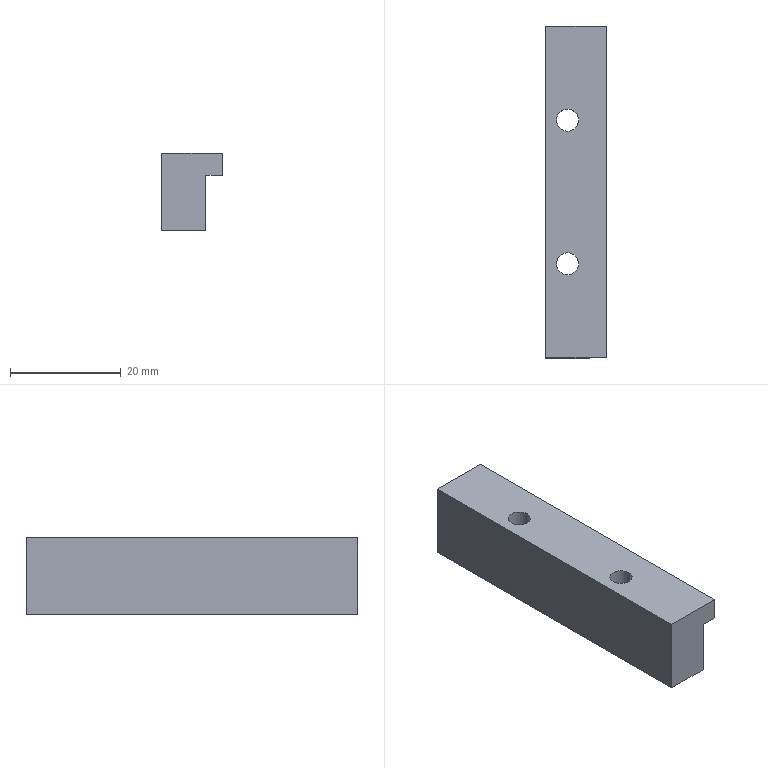Component | NX | 3_RECTANGULAR_GUIDE | 1 solid | 14 faces | box 11 x 60 x 14 mm | volume 6744 mm3 | plane 8 | cylinder 4 | cone 2 | commonest cylinder face diameters 4.2 x2 4 x2
STEP:
#1=CARTESIAN_POINT('',(0.,0.,0.));
#2=DIRECTION('',(0.,0.,1.));
#3=DIRECTION('',(1.,0.,0.));
#4=AXIS2_PLACEMENT_3D('',#1,#2,#3);
#5=CARTESIAN_POINT('',(20.,13.,28.));
#6=VERTEX_POINT('',#5);
#7=CARTESIAN_POINT('',(16.,13.,28.));
#8=VERTEX_POINT('',#7);
#9=CARTESIAN_POINT('',(18.,13.,28.));
#10=DIRECTION('',(0.,0.,-1.));
#11=DIRECTION('',(1.,0.,0.));
#12=AXIS2_PLACEMENT_3D('',#9,#10,#11);
#13=CIRCLE('',#12,2.);
#14=CARTESIAN_POINT('',(25.,-30.,28.));
#15=DIRECTION('',(0.,0.,-1.));
#16=DIRECTION('',(1.,0.,0.));
#17=AXIS2_PLACEMENT_3D('',#14,#15,#16);
#18=PLANE('',#17);
#19=CARTESIAN_POINT('',(-7.,-43.));
#20=DIRECTION('',(1.,0.));
#21=AXIS2_PLACEMENT_2D('',#19,#20);
#22=CIRCLE('',#21,2.);
#23=(GEOMETRIC_REPRESENTATION_CONTEXT(2)PARAMETRIC_REPRESENTATION_CONTEXT()REPRESENTATION_CONTEXT('',''));
#24=DEFINITIONAL_REPRESENTATION('',(#22),#23);
#25=PCURVE('',#18,#24);
#26=CARTESIAN_POINT('',(18.,13.,14.));
#27=DIRECTION('',(-0.,0.,1.));
#28=DIRECTION('',(-1.,0.,-0.));
#29=AXIS2_PLACEMENT_3D('',#26,#27,#28);
#30=CYLINDRICAL_SURFACE('',#29,2.);
#31=CARTESIAN_POINT('',(3.142,14.));
#32=DIRECTION('',(-1.,0.));
#33=VECTOR('',#32,1.);
#34=LINE('',#31,#33);
#35=(GEOMETRIC_REPRESENTATION_CONTEXT(2)PARAMETRIC_REPRESENTATION_CONTEXT()REPRESENTATION_CONTEXT('',''));
#36=DEFINITIONAL_REPRESENTATION('',(#34),#35);
#37=PCURVE('',#30,#36);
#38=SURFACE_CURVE('',#13,(#25,#37),.PCURVE_S1.);
#39=EDGE_CURVE('',#6,#8,#38,.T.);
#40=ORIENTED_EDGE('',*,*,#39,.T.);
#41=CARTESIAN_POINT('',(18.,13.,28.));
#42=DIRECTION('',(0.,0.,-1.));
#43=DIRECTION('',(1.,0.,0.));
#44=AXIS2_PLACEMENT_3D('',#41,#42,#43);
#45=CIRCLE('',#44,2.);
#46=CARTESIAN_POINT('',(-7.,-43.));
#47=DIRECTION('',(1.,0.));
#48=AXIS2_PLACEMENT_2D('',#46,#47);
#49=CIRCLE('',#48,2.);
#50=(GEOMETRIC_REPRESENTATION_CONTEXT(2)PARAMETRIC_REPRESENTATION_CONTEXT()REPRESENTATION_CONTEXT('',''));
#51=DEFINITIONAL_REPRESENTATION('',(#49),#50);
#52=PCURVE('',#18,#51);
#53=CARTESIAN_POINT('',(9.425,14.));
#54=DIRECTION('',(-1.,0.));
#55=VECTOR('',#54,1.);
#56=LINE('',#53,#55);
#57=(GEOMETRIC_REPRESENTATION_CONTEXT(2)PARAMETRIC_REPRESENTATION_CONTEXT()REPRESENTATION_CONTEXT('',''));
#58=DEFINITIONAL_REPRESENTATION('',(#56),#57);
#59=PCURVE('',#30,#58);
#60=SURFACE_CURVE('',#45,(#52,#59),.PCURVE_S1.);
#61=EDGE_CURVE('',#8,#6,#60,.T.);
#62=ORIENTED_EDGE('',*,*,#61,.T.);
#63=EDGE_LOOP('',(#40,#62));
#64=FACE_BOUND('',#63,.T.);
#65=CARTESIAN_POINT('',(20.,-13.,28.));
#66=VERTEX_POINT('',#65);
#67=CARTESIAN_POINT('',(16.,-13.,28.));
#68=VERTEX_POINT('',#67);
#69=CARTESIAN_POINT('',(18.,-13.,28.));
#70=DIRECTION('',(0.,0.,-1.));
#71=DIRECTION('',(1.,0.,0.));
#72=AXIS2_PLACEMENT_3D('',#69,#70,#71);
#73=CIRCLE('',#72,2.);
#74=CARTESIAN_POINT('',(-7.,-17.));
#75=DIRECTION('',(1.,0.));
#76=AXIS2_PLACEMENT_2D('',#74,#75);
#77=CIRCLE('',#76,2.);
#78=(GEOMETRIC_REPRESENTATION_CONTEXT(2)PARAMETRIC_REPRESENTATION_CONTEXT()REPRESENTATION_CONTEXT('',''));
#79=DEFINITIONAL_REPRESENTATION('',(#77),#78);
#80=PCURVE('',#18,#79);
#81=CARTESIAN_POINT('',(18.,-13.,14.));
#82=DIRECTION('',(-0.,0.,1.));
#83=DIRECTION('',(-1.,0.,-0.));
#84=AXIS2_PLACEMENT_3D('',#81,#82,#83);
#85=CYLINDRICAL_SURFACE('',#84,2.);
#86=CARTESIAN_POINT('',(3.142,14.));
#87=DIRECTION('',(-1.,0.));
#88=VECTOR('',#87,1.);
#89=LINE('',#86,#88);
#90=(GEOMETRIC_REPRESENTATION_CONTEXT(2)PARAMETRIC_REPRESENTATION_CONTEXT()REPRESENTATION_CONTEXT('',''));
#91=DEFINITIONAL_REPRESENTATION('',(#89),#90);
#92=PCURVE('',#85,#91);
#93=SURFACE_CURVE('',#73,(#80,#92),.PCURVE_S1.);
#94=EDGE_CURVE('',#66,#68,#93,.T.);
#95=ORIENTED_EDGE('',*,*,#94,.T.);
#96=CARTESIAN_POINT('',(18.,-13.,28.));
#97=DIRECTION('',(0.,0.,-1.));
#98=DIRECTION('',(1.,0.,0.));
#99=AXIS2_PLACEMENT_3D('',#96,#97,#98);
#100=CIRCLE('',#99,2.);
#101=CARTESIAN_POINT('',(-7.,-17.));
#102=DIRECTION('',(1.,0.));
#103=AXIS2_PLACEMENT_2D('',#101,#102);
#104=CIRCLE('',#103,2.);
#105=(GEOMETRIC_REPRESENTATION_CONTEXT(2)PARAMETRIC_REPRESENTATION_CONTEXT()REPRESENTATION_CONTEXT('',''));
#106=DEFINITIONAL_REPRESENTATION('',(#104),#105);
#107=PCURVE('',#18,#106);
#108=CARTESIAN_POINT('',(9.425,14.));
#109=DIRECTION('',(-1.,0.));
#110=VECTOR('',#109,1.);
#111=LINE('',#108,#110);
#112=(GEOMETRIC_REPRESENTATION_CONTEXT(2)PARAMETRIC_REPRESENTATION_CONTEXT()REPRESENTATION_CONTEXT('',''));
#113=DEFINITIONAL_REPRESENTATION('',(#111),#112);
#114=PCURVE('',#85,#113);
#115=SURFACE_CURVE('',#100,(#107,#114),.PCURVE_S1.);
#116=EDGE_CURVE('',#68,#66,#115,.T.);
#117=ORIENTED_EDGE('',*,*,#116,.T.);
#118=EDGE_LOOP('',(#95,#117));
#119=FACE_BOUND('',#118,.T.);
#120=CARTESIAN_POINT('',(25.,30.,28.));
#121=VERTEX_POINT('',#120);
#122=CARTESIAN_POINT('',(14.,30.,28.));
#123=VERTEX_POINT('',#122);
#124=CARTESIAN_POINT('',(25.,30.,28.));
#125=DIRECTION('',(-1.,0.,0.));
#126=VECTOR('',#125,1.);
#127=LINE('',#124,#126);
#128=CARTESIAN_POINT('',(0.,-60.));
#129=DIRECTION('',(-1.,0.));
#130=VECTOR('',#129,1.);
#131=LINE('',#128,#130);
#132=(GEOMETRIC_REPRESENTATION_CONTEXT(2)PARAMETRIC_REPRESENTATION_CONTEXT()REPRESENTATION_CONTEXT('',''));
#133=DEFINITIONAL_REPRESENTATION('',(#131),#132);
#134=PCURVE('',#18,#133);
#135=CARTESIAN_POINT('',(14.,30.,28.));
#136=DIRECTION('',(0.,-1.,0.));
#137=DIRECTION('',(-1.,0.,0.));
#138=AXIS2_PLACEMENT_3D('',#135,#136,#137);
#139=PLANE('',#138);
#140=CARTESIAN_POINT('',(-11.,0.));
#141=DIRECTION('',(1.,0.));
#142=VECTOR('',#141,1.);
#143=LINE('',#140,#142);
#144=(GEOMETRIC_REPRESENTATION_CONTEXT(2)PARAMETRIC_REPRESENTATION_CONTEXT()REPRESENTATION_CONTEXT('',''));
#145=DEFINITIONAL_REPRESENTATION('',(#143),#144);
#146=PCURVE('',#139,#145);
#147=SURFACE_CURVE('',#127,(#134,#146),.PCURVE_S1.);
#148=EDGE_CURVE('',#121,#123,#147,.T.);
#149=ORIENTED_EDGE('',*,*,#148,.T.);
#150=CARTESIAN_POINT('',(14.,-30.,28.));
#151=VERTEX_POINT('',#150);
#152=CARTESIAN_POINT('',(14.,-30.,28.));
#153=DIRECTION('',(0.,1.,0.));
#154=VECTOR('',#153,1.);
#155=LINE('',#152,#154);
#156=CARTESIAN_POINT('',(-11.,0.));
#157=DIRECTION('',(0.,-1.));
#158=VECTOR('',#157,1.);
#159=LINE('',#156,#158);
#160=(GEOMETRIC_REPRESENTATION_CONTEXT(2)PARAMETRIC_REPRESENTATION_CONTEXT()REPRESENTATION_CONTEXT('',''));
#161=DEFINITIONAL_REPRESENTATION('',(#159),#160);
#162=PCURVE('',#18,#161);
#163=CARTESIAN_POINT('',(14.,-30.,24.));
#164=DIRECTION('',(1.,0.,0.));
#165=DIRECTION('',(0.,-1.,0.));
#166=AXIS2_PLACEMENT_3D('',#163,#164,#165);
#167=PLANE('',#166);
#168=CARTESIAN_POINT('',(0.,-4.));
#169=DIRECTION('',(-1.,0.));
#170=VECTOR('',#169,1.);
#171=LINE('',#168,#170);
#172=(GEOMETRIC_REPRESENTATION_CONTEXT(2)PARAMETRIC_REPRESENTATION_CONTEXT()REPRESENTATION_CONTEXT('',''));
#173=DEFINITIONAL_REPRESENTATION('',(#171),#172);
#174=PCURVE('',#167,#173);
#175=SURFACE_CURVE('',#155,(#162,#174),.PCURVE_S1.);
#176=EDGE_CURVE('',#151,#123,#175,.T.);
#177=ORIENTED_EDGE('',*,*,#176,.F.);
#178=CARTESIAN_POINT('',(25.,-30.,28.));
#179=VERTEX_POINT('',#178);
#180=CARTESIAN_POINT('',(25.,-30.,28.));
#181=DIRECTION('',(-1.,0.,0.));
#182=VECTOR('',#181,1.);
#183=LINE('',#180,#182);
#184=CARTESIAN_POINT('',(0.,0.));
#185=DIRECTION('',(-1.,0.));
#186=VECTOR('',#185,1.);
#187=LINE('',#184,#186);
#188=(GEOMETRIC_REPRESENTATION_CONTEXT(2)PARAMETRIC_REPRESENTATION_CONTEXT()REPRESENTATION_CONTEXT('',''));
#189=DEFINITIONAL_REPRESENTATION('',(#187),#188);
#190=PCURVE('',#18,#189);
#191=CARTESIAN_POINT('',(14.,-30.,28.));
#192=DIRECTION('',(0.,-1.,0.));
#193=DIRECTION('',(-1.,0.,0.));
#194=AXIS2_PLACEMENT_3D('',#191,#192,#193);
#195=PLANE('',#194);
#196=CARTESIAN_POINT('',(-11.,0.));
#197=DIRECTION('',(1.,0.));
#198=VECTOR('',#197,1.);
#199=LINE('',#196,#198);
#200=(GEOMETRIC_REPRESENTATION_CONTEXT(2)PARAMETRIC_REPRESENTATION_CONTEXT()REPRESENTATION_CONTEXT('',''));
#201=DEFINITIONAL_REPRESENTATION('',(#199),#200);
#202=PCURVE('',#195,#201);
#203=SURFACE_CURVE('',#183,(#190,#202),.PCURVE_S1.);
#204=EDGE_CURVE('',#179,#151,#203,.T.);
#205=ORIENTED_EDGE('',*,*,#204,.F.);
#206=CARTESIAN_POINT('',(25.,-30.,28.));
#207=DIRECTION('',(0.,1.,0.));
#208=VECTOR('',#207,1.);
#209=LINE('',#206,#208);
#210=CARTESIAN_POINT('',(0.,0.));
#211=DIRECTION('',(0.,-1.));
#212=VECTOR('',#211,1.);
#213=LINE('',#210,#212);
#214=(GEOMETRIC_REPRESENTATION_CONTEXT(2)PARAMETRIC_REPRESENTATION_CONTEXT()REPRESENTATION_CONTEXT('',''));
#215=DEFINITIONAL_REPRESENTATION('',(#213),#214);
#216=PCURVE('',#18,#215);
#217=CARTESIAN_POINT('',(25.,-30.,24.));
#218=DIRECTION('',(-1.,0.,0.));
#219=DIRECTION('',(0.,1.,0.));
#220=AXIS2_PLACEMENT_3D('',#217,#218,#219);
#221=PLANE('',#220);
#222=CARTESIAN_POINT('',(0.,-4.));
#223=DIRECTION('',(1.,0.));
#224=VECTOR('',#223,1.);
#225=LINE('',#222,#224);
#226=(GEOMETRIC_REPRESENTATION_CONTEXT(2)PARAMETRIC_REPRESENTATION_CONTEXT()REPRESENTATION_CONTEXT('',''));
#227=DEFINITIONAL_REPRESENTATION('',(#225),#226);
#228=PCURVE('',#221,#227);
#229=SURFACE_CURVE('',#209,(#216,#228),.PCURVE_S1.);
#230=EDGE_CURVE('',#179,#121,#229,.T.);
#231=ORIENTED_EDGE('',*,*,#230,.T.);
#232=EDGE_LOOP('',(#149,#177,#205,#231));
#233=FACE_BOUND('',#232,.T.);
#234=ADVANCED_FACE('',(#64,#119,#233),#18,.F.);
#235=CARTESIAN_POINT('',(14.,30.,14.));
#236=VERTEX_POINT('',#235);
#237=CARTESIAN_POINT('',(14.,30.,24.));
#238=DIRECTION('',(0.,0.,-1.));
#239=VECTOR('',#238,1.);
#240=LINE('',#237,#239);
#241=CARTESIAN_POINT('',(-60.,0.));
#242=DIRECTION('',(0.,1.));
#243=VECTOR('',#242,1.);
#244=LINE('',#241,#243);
#245=(GEOMETRIC_REPRESENTATION_CONTEXT(2)PARAMETRIC_REPRESENTATION_CONTEXT()REPRESENTATION_CONTEXT('',''));
#246=DEFINITIONAL_REPRESENTATION('',(#244),#245);
#247=PCURVE('',#167,#246);
#248=CARTESIAN_POINT('',(0.,4.));
#249=DIRECTION('',(0.,1.));
#250=VECTOR('',#249,1.);
#251=LINE('',#248,#250);
#252=(GEOMETRIC_REPRESENTATION_CONTEXT(2)PARAMETRIC_REPRESENTATION_CONTEXT()REPRESENTATION_CONTEXT('',''));
#253=DEFINITIONAL_REPRESENTATION('',(#251),#252);
#254=PCURVE('',#139,#253);
#255=SURFACE_CURVE('',#240,(#247,#254),.PCURVE_S1.);
#256=EDGE_CURVE('',#123,#236,#255,.T.);
#257=ORIENTED_EDGE('',*,*,#256,.T.);
#258=CARTESIAN_POINT('',(14.,-30.,14.));
#259=VERTEX_POINT('',#258);
#260=CARTESIAN_POINT('',(14.,-30.,14.));
#261=DIRECTION('',(0.,1.,0.));
#262=VECTOR('',#261,1.);
#263=LINE('',#260,#262);
#264=CARTESIAN_POINT('',(0.,10.));
#265=DIRECTION('',(-1.,0.));
#266=VECTOR('',#265,1.);
#267=LINE('',#264,#266);
#268=(GEOMETRIC_REPRESENTATION_CONTEXT(2)PARAMETRIC_REPRESENTATION_CONTEXT()REPRESENTATION_CONTEXT('',''));
#269=DEFINITIONAL_REPRESENTATION('',(#267),#268);
#270=PCURVE('',#167,#269);
#271=CARTESIAN_POINT('',(14.,-30.,14.));
#272=DIRECTION('',(-0.,0.,1.));
#273=DIRECTION('',(-1.,0.,-0.));
#274=AXIS2_PLACEMENT_3D('',#271,#272,#273);
#275=PLANE('',#274);
#276=CARTESIAN_POINT('',(0.,0.));
#277=DIRECTION('',(0.,-1.));
#278=VECTOR('',#277,1.);
#279=LINE('',#276,#278);
#280=(GEOMETRIC_REPRESENTATION_CONTEXT(2)PARAMETRIC_REPRESENTATION_CONTEXT()REPRESENTATION_CONTEXT('',''));
#281=DEFINITIONAL_REPRESENTATION('',(#279),#280);
#282=PCURVE('',#275,#281);
#283=SURFACE_CURVE('',#263,(#270,#282),.PCURVE_S1.);
#284=EDGE_CURVE('',#259,#236,#283,.T.);
#285=ORIENTED_EDGE('',*,*,#284,.F.);
#286=CARTESIAN_POINT('',(14.,-30.,28.));
#287=DIRECTION('',(0.,0.,-1.));
#288=VECTOR('',#287,1.);
#289=LINE('',#286,#288);
#290=CARTESIAN_POINT('',(0.,-4.));
#291=DIRECTION('',(0.,1.));
#292=VECTOR('',#291,1.);
#293=LINE('',#290,#292);
#294=(GEOMETRIC_REPRESENTATION_CONTEXT(2)PARAMETRIC_REPRESENTATION_CONTEXT()REPRESENTATION_CONTEXT('',''));
#295=DEFINITIONAL_REPRESENTATION('',(#293),#294);
#296=PCURVE('',#167,#295);
#297=CARTESIAN_POINT('',(0.,0.));
#298=DIRECTION('',(0.,1.));
#299=VECTOR('',#298,1.);
#300=LINE('',#297,#299);
#301=(GEOMETRIC_REPRESENTATION_CONTEXT(2)PARAMETRIC_REPRESENTATION_CONTEXT()REPRESENTATION_CONTEXT('',''));
#302=DEFINITIONAL_REPRESENTATION('',(#300),#301);
#303=PCURVE('',#195,#302);
#304=SURFACE_CURVE('',#289,(#296,#303),.PCURVE_S1.);
#305=EDGE_CURVE('',#151,#259,#304,.T.);
#306=ORIENTED_EDGE('',*,*,#305,.F.);
#307=ORIENTED_EDGE('',*,*,#176,.T.);
#308=EDGE_LOOP('',(#257,#285,#306,#307));
#309=FACE_BOUND('',#308,.T.);
#310=ADVANCED_FACE('',(#309),#167,.F.);
#311=CARTESIAN_POINT('',(16.,13.,14.));
#312=VERTEX_POINT('',#311);
#313=CARTESIAN_POINT('',(18.,13.,14.));
#314=DIRECTION('',(-0.,0.,1.));
#315=DIRECTION('',(-1.,0.,-0.));
#316=AXIS2_PLACEMENT_3D('',#313,#314,#315);
#317=CIRCLE('',#316,2.);
#318=CARTESIAN_POINT('',(-4.,-43.));
#319=DIRECTION('',(1.,0.));
#320=AXIS2_PLACEMENT_2D('',#318,#319);
#321=CIRCLE('',#320,2.);
#322=(GEOMETRIC_REPRESENTATION_CONTEXT(2)PARAMETRIC_REPRESENTATION_CONTEXT()REPRESENTATION_CONTEXT('',''));
#323=DEFINITIONAL_REPRESENTATION('',(#321),#322);
#324=PCURVE('',#275,#323);
#325=CARTESIAN_POINT('',(0.,0.));
#326=DIRECTION('',(1.,0.));
#327=VECTOR('',#326,1.);
#328=LINE('',#325,#327);
#329=(GEOMETRIC_REPRESENTATION_CONTEXT(2)PARAMETRIC_REPRESENTATION_CONTEXT()REPRESENTATION_CONTEXT('',''));
#330=DEFINITIONAL_REPRESENTATION('',(#328),#329);
#331=PCURVE('',#30,#330);
#332=SURFACE_CURVE('',#317,(#324,#331),.PCURVE_S1.);
#333=EDGE_CURVE('',#312,#312,#332,.T.);
#334=ORIENTED_EDGE('',*,*,#333,.T.);
#335=EDGE_LOOP('',(#334));
#336=FACE_BOUND('',#335,.T.);
#337=CARTESIAN_POINT('',(16.,-13.,14.));
#338=VERTEX_POINT('',#337);
#339=CARTESIAN_POINT('',(18.,-13.,14.));
#340=DIRECTION('',(-0.,0.,1.));
#341=DIRECTION('',(-1.,0.,-0.));
#342=AXIS2_PLACEMENT_3D('',#339,#340,#341);
#343=CIRCLE('',#342,2.);
#344=CARTESIAN_POINT('',(-4.,-17.));
#345=DIRECTION('',(1.,0.));
#346=AXIS2_PLACEMENT_2D('',#344,#345);
#347=CIRCLE('',#346,2.);
#348=(GEOMETRIC_REPRESENTATION_CONTEXT(2)PARAMETRIC_REPRESENTATION_CONTEXT()REPRESENTATION_CONTEXT('',''));
#349=DEFINITIONAL_REPRESENTATION('',(#347),#348);
#350=PCURVE('',#275,#349);
#351=CARTESIAN_POINT('',(0.,0.));
#352=DIRECTION('',(1.,0.));
#353=VECTOR('',#352,1.);
#354=LINE('',#351,#353);
#355=(GEOMETRIC_REPRESENTATION_CONTEXT(2)PARAMETRIC_REPRESENTATION_CONTEXT()REPRESENTATION_CONTEXT('',''));
#356=DEFINITIONAL_REPRESENTATION('',(#354),#355);
#357=PCURVE('',#85,#356);
#358=SURFACE_CURVE('',#343,(#350,#357),.PCURVE_S1.);
#359=EDGE_CURVE('',#338,#338,#358,.T.);
#360=ORIENTED_EDGE('',*,*,#359,.T.);
#361=EDGE_LOOP('',(#360));
#362=FACE_BOUND('',#361,.T.);
#363=CARTESIAN_POINT('',(15.9,22.,14.));
#364=VERTEX_POINT('',#363);
#365=CARTESIAN_POINT('',(18.,22.,14.));
#366=DIRECTION('',(-0.,0.,1.));
#367=DIRECTION('',(-1.,0.,-0.));
#368=AXIS2_PLACEMENT_3D('',#365,#366,#367);
#369=CIRCLE('',#368,2.1);
#370=CARTESIAN_POINT('',(-4.,-52.));
#371=DIRECTION('',(1.,0.));
#372=AXIS2_PLACEMENT_2D('',#370,#371);
#373=CIRCLE('',#372,2.1);
#374=(GEOMETRIC_REPRESENTATION_CONTEXT(2)PARAMETRIC_REPRESENTATION_CONTEXT()REPRESENTATION_CONTEXT('',''));
#375=DEFINITIONAL_REPRESENTATION('',(#373),#374);
#376=PCURVE('',#275,#375);
#377=CARTESIAN_POINT('',(18.,22.,14.));
#378=DIRECTION('',(-0.,0.,1.));
#379=DIRECTION('',(-1.,0.,-0.));
#380=AXIS2_PLACEMENT_3D('',#377,#378,#379);
#381=CYLINDRICAL_SURFACE('',#380,2.1);
#382=CARTESIAN_POINT('',(0.,0.));
#383=DIRECTION('',(1.,0.));
#384=VECTOR('',#383,1.);
#385=LINE('',#382,#384);
#386=(GEOMETRIC_REPRESENTATION_CONTEXT(2)PARAMETRIC_REPRESENTATION_CONTEXT()REPRESENTATION_CONTEXT('',''));
#387=DEFINITIONAL_REPRESENTATION('',(#385),#386);
#388=PCURVE('',#381,#387);
#389=SURFACE_CURVE('',#369,(#376,#388),.PCURVE_S1.);
#390=EDGE_CURVE('',#364,#364,#389,.T.);
#391=ORIENTED_EDGE('',*,*,#390,.T.);
#392=EDGE_LOOP('',(#391));
#393=FACE_BOUND('',#392,.T.);
#394=CARTESIAN_POINT('',(15.9,-22.,14.));
#395=VERTEX_POINT('',#394);
#396=CARTESIAN_POINT('',(18.,-22.,14.));
#397=DIRECTION('',(-0.,0.,1.));
#398=DIRECTION('',(-1.,0.,-0.));
#399=AXIS2_PLACEMENT_3D('',#396,#397,#398);
#400=CIRCLE('',#399,2.1);
#401=CARTESIAN_POINT('',(-4.,-8.));
#402=DIRECTION('',(1.,0.));
#403=AXIS2_PLACEMENT_2D('',#401,#402);
#404=CIRCLE('',#403,2.1);
#405=(GEOMETRIC_REPRESENTATION_CONTEXT(2)PARAMETRIC_REPRESENTATION_CONTEXT()REPRESENTATION_CONTEXT('',''));
#406=DEFINITIONAL_REPRESENTATION('',(#404),#405);
#407=PCURVE('',#275,#406);
#408=CARTESIAN_POINT('',(18.,-22.,14.));
#409=DIRECTION('',(-0.,0.,1.));
#410=DIRECTION('',(-1.,0.,-0.));
#411=AXIS2_PLACEMENT_3D('',#408,#409,#410);
#412=CYLINDRICAL_SURFACE('',#411,2.1);
#413=CARTESIAN_POINT('',(0.,0.));
#414=DIRECTION('',(1.,0.));
#415=VECTOR('',#414,1.);
#416=LINE('',#413,#415);
#417=(GEOMETRIC_REPRESENTATION_CONTEXT(2)PARAMETRIC_REPRESENTATION_CONTEXT()REPRESENTATION_CONTEXT('',''));
#418=DEFINITIONAL_REPRESENTATION('',(#416),#417);
#419=PCURVE('',#412,#418);
#420=SURFACE_CURVE('',#400,(#407,#419),.PCURVE_S1.);
#421=EDGE_CURVE('',#395,#395,#420,.T.);
#422=ORIENTED_EDGE('',*,*,#421,.T.);
#423=EDGE_LOOP('',(#422));
#424=FACE_BOUND('',#423,.T.);
#425=CARTESIAN_POINT('',(22.,30.,14.));
#426=VERTEX_POINT('',#425);
#427=CARTESIAN_POINT('',(14.,30.,14.));
#428=DIRECTION('',(1.,0.,0.));
#429=VECTOR('',#428,1.);
#430=LINE('',#427,#429);
#431=CARTESIAN_POINT('',(0.,-60.));
#432=DIRECTION('',(-1.,0.));
#433=VECTOR('',#432,1.);
#434=LINE('',#431,#433);
#435=(GEOMETRIC_REPRESENTATION_CONTEXT(2)PARAMETRIC_REPRESENTATION_CONTEXT()REPRESENTATION_CONTEXT('',''));
#436=DEFINITIONAL_REPRESENTATION('',(#434),#435);
#437=PCURVE('',#275,#436);
#438=CARTESIAN_POINT('',(0.,14.));
#439=DIRECTION('',(-1.,-0.));
#440=VECTOR('',#439,1.);
#441=LINE('',#438,#440);
#442=(GEOMETRIC_REPRESENTATION_CONTEXT(2)PARAMETRIC_REPRESENTATION_CONTEXT()REPRESENTATION_CONTEXT('',''));
#443=DEFINITIONAL_REPRESENTATION('',(#441),#442);
#444=PCURVE('',#139,#443);
#445=SURFACE_CURVE('',#430,(#437,#444),.PCURVE_S1.);
#446=EDGE_CURVE('',#236,#426,#445,.T.);
#447=ORIENTED_EDGE('',*,*,#446,.T.);
#448=CARTESIAN_POINT('',(22.,-30.,14.));
#449=VERTEX_POINT('',#448);
#450=CARTESIAN_POINT('',(22.,-30.,14.));
#451=DIRECTION('',(0.,1.,0.));
#452=VECTOR('',#451,1.);
#453=LINE('',#450,#452);
#454=CARTESIAN_POINT('',(-8.,0.));
#455=DIRECTION('',(0.,-1.));
#456=VECTOR('',#455,1.);
#457=LINE('',#454,#456);
#458=(GEOMETRIC_REPRESENTATION_CONTEXT(2)PARAMETRIC_REPRESENTATION_CONTEXT()REPRESENTATION_CONTEXT('',''));
#459=DEFINITIONAL_REPRESENTATION('',(#457),#458);
#460=PCURVE('',#275,#459);
#461=CARTESIAN_POINT('',(22.,-30.,14.));
#462=DIRECTION('',(-1.,0.,-0.));
#463=DIRECTION('',(0.,0.,-1.));
#464=AXIS2_PLACEMENT_3D('',#461,#462,#463);
#465=PLANE('',#464);
#466=CARTESIAN_POINT('',(0.,0.));
#467=DIRECTION('',(0.,-1.));
#468=VECTOR('',#467,1.);
#469=LINE('',#466,#468);
#470=(GEOMETRIC_REPRESENTATION_CONTEXT(2)PARAMETRIC_REPRESENTATION_CONTEXT()REPRESENTATION_CONTEXT('',''));
#471=DEFINITIONAL_REPRESENTATION('',(#469),#470);
#472=PCURVE('',#465,#471);
#473=SURFACE_CURVE('',#453,(#460,#472),.PCURVE_S1.);
#474=EDGE_CURVE('',#449,#426,#473,.T.);
#475=ORIENTED_EDGE('',*,*,#474,.F.);
#476=CARTESIAN_POINT('',(14.,-30.,14.));
#477=DIRECTION('',(1.,0.,0.));
#478=VECTOR('',#477,1.);
#479=LINE('',#476,#478);
#480=CARTESIAN_POINT('',(0.,0.));
#481=DIRECTION('',(-1.,0.));
#482=VECTOR('',#481,1.);
#483=LINE('',#480,#482);
#484=(GEOMETRIC_REPRESENTATION_CONTEXT(2)PARAMETRIC_REPRESENTATION_CONTEXT()REPRESENTATION_CONTEXT('',''));
#485=DEFINITIONAL_REPRESENTATION('',(#483),#484);
#486=PCURVE('',#275,#485);
#487=CARTESIAN_POINT('',(0.,14.));
#488=DIRECTION('',(-1.,-0.));
#489=VECTOR('',#488,1.);
#490=LINE('',#487,#489);
#491=(GEOMETRIC_REPRESENTATION_CONTEXT(2)PARAMETRIC_REPRESENTATION_CONTEXT()REPRESENTATION_CONTEXT('',''));
#492=DEFINITIONAL_REPRESENTATION('',(#490),#491);
#493=PCURVE('',#195,#492);
#494=SURFACE_CURVE('',#479,(#486,#493),.PCURVE_S1.);
#495=EDGE_CURVE('',#259,#449,#494,.T.);
#496=ORIENTED_EDGE('',*,*,#495,.F.);
#497=ORIENTED_EDGE('',*,*,#284,.T.);
#498=EDGE_LOOP('',(#447,#475,#496,#497));
#499=FACE_BOUND('',#498,.T.);
#500=ADVANCED_FACE('',(#336,#362,#393,#424,#499),#275,.F.);
#501=CARTESIAN_POINT('',(22.,30.,24.));
#502=VERTEX_POINT('',#501);
#503=CARTESIAN_POINT('',(22.,30.,14.));
#504=DIRECTION('',(-0.,0.,1.));
#505=VECTOR('',#504,1.);
#506=LINE('',#503,#505);
#507=CARTESIAN_POINT('',(0.,-60.));
#508=DIRECTION('',(-1.,0.));
#509=VECTOR('',#508,1.);
#510=LINE('',#507,#509);
#511=(GEOMETRIC_REPRESENTATION_CONTEXT(2)PARAMETRIC_REPRESENTATION_CONTEXT()REPRESENTATION_CONTEXT('',''));
#512=DEFINITIONAL_REPRESENTATION('',(#510),#511);
#513=PCURVE('',#465,#512);
#514=CARTESIAN_POINT('',(-8.,14.));
#515=DIRECTION('',(0.,-1.));
#516=VECTOR('',#515,1.);
#517=LINE('',#514,#516);
#518=(GEOMETRIC_REPRESENTATION_CONTEXT(2)PARAMETRIC_REPRESENTATION_CONTEXT()REPRESENTATION_CONTEXT('',''));
#519=DEFINITIONAL_REPRESENTATION('',(#517),#518);
#520=PCURVE('',#139,#519);
#521=SURFACE_CURVE('',#506,(#513,#520),.PCURVE_S1.);
#522=EDGE_CURVE('',#426,#502,#521,.T.);
#523=ORIENTED_EDGE('',*,*,#522,.T.);
#524=CARTESIAN_POINT('',(22.,-30.,24.));
#525=VERTEX_POINT('',#524);
#526=CARTESIAN_POINT('',(22.,-30.,24.));
#527=DIRECTION('',(0.,1.,0.));
#528=VECTOR('',#527,1.);
#529=LINE('',#526,#528);
#530=CARTESIAN_POINT('',(-10.,0.));
#531=DIRECTION('',(0.,-1.));
#532=VECTOR('',#531,1.);
#533=LINE('',#530,#532);
#534=(GEOMETRIC_REPRESENTATION_CONTEXT(2)PARAMETRIC_REPRESENTATION_CONTEXT()REPRESENTATION_CONTEXT('',''));
#535=DEFINITIONAL_REPRESENTATION('',(#533),#534);
#536=PCURVE('',#465,#535);
#537=CARTESIAN_POINT('',(22.,-30.,24.));
#538=DIRECTION('',(-0.,0.,1.));
#539=DIRECTION('',(-1.,0.,-0.));
#540=AXIS2_PLACEMENT_3D('',#537,#538,#539);
#541=PLANE('',#540);
#542=CARTESIAN_POINT('',(0.,0.));
#543=DIRECTION('',(0.,-1.));
#544=VECTOR('',#543,1.);
#545=LINE('',#542,#544);
#546=(GEOMETRIC_REPRESENTATION_CONTEXT(2)PARAMETRIC_REPRESENTATION_CONTEXT()REPRESENTATION_CONTEXT('',''));
#547=DEFINITIONAL_REPRESENTATION('',(#545),#546);
#548=PCURVE('',#541,#547);
#549=SURFACE_CURVE('',#529,(#536,#548),.PCURVE_S1.);
#550=EDGE_CURVE('',#525,#502,#549,.T.);
#551=ORIENTED_EDGE('',*,*,#550,.F.);
#552=CARTESIAN_POINT('',(22.,-30.,14.));
#553=DIRECTION('',(-0.,0.,1.));
#554=VECTOR('',#553,1.);
#555=LINE('',#552,#554);
#556=CARTESIAN_POINT('',(0.,0.));
#557=DIRECTION('',(-1.,0.));
#558=VECTOR('',#557,1.);
#559=LINE('',#556,#558);
#560=(GEOMETRIC_REPRESENTATION_CONTEXT(2)PARAMETRIC_REPRESENTATION_CONTEXT()REPRESENTATION_CONTEXT('',''));
#561=DEFINITIONAL_REPRESENTATION('',(#559),#560);
#562=PCURVE('',#465,#561);
#563=CARTESIAN_POINT('',(-8.,14.));
#564=DIRECTION('',(0.,-1.));
#565=VECTOR('',#564,1.);
#566=LINE('',#563,#565);
#567=(GEOMETRIC_REPRESENTATION_CONTEXT(2)PARAMETRIC_REPRESENTATION_CONTEXT()REPRESENTATION_CONTEXT('',''));
#568=DEFINITIONAL_REPRESENTATION('',(#566),#567);
#569=PCURVE('',#195,#568);
#570=SURFACE_CURVE('',#555,(#562,#569),.PCURVE_S1.);
#571=EDGE_CURVE('',#449,#525,#570,.T.);
#572=ORIENTED_EDGE('',*,*,#571,.F.);
#573=ORIENTED_EDGE('',*,*,#474,.T.);
#574=EDGE_LOOP('',(#523,#551,#572,#573));
#575=FACE_BOUND('',#574,.T.);
#576=ADVANCED_FACE('',(#575),#465,.F.);
#577=CARTESIAN_POINT('',(25.,30.,24.));
#578=VERTEX_POINT('',#577);
#579=CARTESIAN_POINT('',(22.,30.,24.));
#580=DIRECTION('',(1.,0.,0.));
#581=VECTOR('',#580,1.);
#582=LINE('',#579,#581);
#583=CARTESIAN_POINT('',(0.,-60.));
#584=DIRECTION('',(-1.,0.));
#585=VECTOR('',#584,1.);
#586=LINE('',#583,#585);
#587=(GEOMETRIC_REPRESENTATION_CONTEXT(2)PARAMETRIC_REPRESENTATION_CONTEXT()REPRESENTATION_CONTEXT('',''));
#588=DEFINITIONAL_REPRESENTATION('',(#586),#587);
#589=PCURVE('',#541,#588);
#590=CARTESIAN_POINT('',(-8.,4.));
#591=DIRECTION('',(-1.,-0.));
#592=VECTOR('',#591,1.);
#593=LINE('',#590,#592);
#594=(GEOMETRIC_REPRESENTATION_CONTEXT(2)PARAMETRIC_REPRESENTATION_CONTEXT()REPRESENTATION_CONTEXT('',''));
#595=DEFINITIONAL_REPRESENTATION('',(#593),#594);
#596=PCURVE('',#139,#595);
#597=SURFACE_CURVE('',#582,(#589,#596),.PCURVE_S1.);
#598=EDGE_CURVE('',#502,#578,#597,.T.);
#599=ORIENTED_EDGE('',*,*,#598,.T.);
#600=CARTESIAN_POINT('',(25.,-30.,24.));
#601=VERTEX_POINT('',#600);
#602=CARTESIAN_POINT('',(25.,-30.,24.));
#603=DIRECTION('',(0.,1.,0.));
#604=VECTOR('',#603,1.);
#605=LINE('',#602,#604);
#606=CARTESIAN_POINT('',(-3.,0.));
#607=DIRECTION('',(0.,-1.));
#608=VECTOR('',#607,1.);
#609=LINE('',#606,#608);
#610=(GEOMETRIC_REPRESENTATION_CONTEXT(2)PARAMETRIC_REPRESENTATION_CONTEXT()REPRESENTATION_CONTEXT('',''));
#611=DEFINITIONAL_REPRESENTATION('',(#609),#610);
#612=PCURVE('',#541,#611);
#613=CARTESIAN_POINT('',(0.,0.));
#614=DIRECTION('',(1.,0.));
#615=VECTOR('',#614,1.);
#616=LINE('',#613,#615);
#617=(GEOMETRIC_REPRESENTATION_CONTEXT(2)PARAMETRIC_REPRESENTATION_CONTEXT()REPRESENTATION_CONTEXT('',''));
#618=DEFINITIONAL_REPRESENTATION('',(#616),#617);
#619=PCURVE('',#221,#618);
#620=SURFACE_CURVE('',#605,(#612,#619),.PCURVE_S1.);
#621=EDGE_CURVE('',#601,#578,#620,.T.);
#622=ORIENTED_EDGE('',*,*,#621,.F.);
#623=CARTESIAN_POINT('',(22.,-30.,24.));
#624=DIRECTION('',(1.,0.,0.));
#625=VECTOR('',#624,1.);
#626=LINE('',#623,#625);
#627=CARTESIAN_POINT('',(0.,0.));
#628=DIRECTION('',(-1.,0.));
#629=VECTOR('',#628,1.);
#630=LINE('',#627,#629);
#631=(GEOMETRIC_REPRESENTATION_CONTEXT(2)PARAMETRIC_REPRESENTATION_CONTEXT()REPRESENTATION_CONTEXT('',''));
#632=DEFINITIONAL_REPRESENTATION('',(#630),#631);
#633=PCURVE('',#541,#632);
#634=CARTESIAN_POINT('',(-8.,4.));
#635=DIRECTION('',(-1.,-0.));
#636=VECTOR('',#635,1.);
#637=LINE('',#634,#636);
#638=(GEOMETRIC_REPRESENTATION_CONTEXT(2)PARAMETRIC_REPRESENTATION_CONTEXT()REPRESENTATION_CONTEXT('',''));
#639=DEFINITIONAL_REPRESENTATION('',(#637),#638);
#640=PCURVE('',#195,#639);
#641=SURFACE_CURVE('',#626,(#633,#640),.PCURVE_S1.);
#642=EDGE_CURVE('',#525,#601,#641,.T.);
#643=ORIENTED_EDGE('',*,*,#642,.F.);
#644=ORIENTED_EDGE('',*,*,#550,.T.);
#645=EDGE_LOOP('',(#599,#622,#643,#644));
#646=FACE_BOUND('',#645,.T.);
#647=ADVANCED_FACE('',(#646),#541,.F.);
#648=CARTESIAN_POINT('',(25.,30.,24.));
#649=DIRECTION('',(0.,0.,1.));
#650=VECTOR('',#649,1.);
#651=LINE('',#648,#650);
#652=CARTESIAN_POINT('',(60.,0.));
#653=DIRECTION('',(0.,-1.));
#654=VECTOR('',#653,1.);
#655=LINE('',#652,#654);
#656=(GEOMETRIC_REPRESENTATION_CONTEXT(2)PARAMETRIC_REPRESENTATION_CONTEXT()REPRESENTATION_CONTEXT('',''));
#657=DEFINITIONAL_REPRESENTATION('',(#655),#656);
#658=PCURVE('',#221,#657);
#659=CARTESIAN_POINT('',(-11.,4.));
#660=DIRECTION('',(0.,-1.));
#661=VECTOR('',#660,1.);
#662=LINE('',#659,#661);
#663=(GEOMETRIC_REPRESENTATION_CONTEXT(2)PARAMETRIC_REPRESENTATION_CONTEXT()REPRESENTATION_CONTEXT('',''));
#664=DEFINITIONAL_REPRESENTATION('',(#662),#663);
#665=PCURVE('',#139,#664);
#666=SURFACE_CURVE('',#651,(#658,#665),.PCURVE_S1.);
#667=EDGE_CURVE('',#578,#121,#666,.T.);
#668=ORIENTED_EDGE('',*,*,#667,.T.);
#669=ORIENTED_EDGE('',*,*,#230,.F.);
#670=CARTESIAN_POINT('',(25.,-30.,24.));
#671=DIRECTION('',(0.,0.,1.));
#672=VECTOR('',#671,1.);
#673=LINE('',#670,#672);
#674=CARTESIAN_POINT('',(0.,0.));
#675=DIRECTION('',(0.,-1.));
#676=VECTOR('',#675,1.);
#677=LINE('',#674,#676);
#678=(GEOMETRIC_REPRESENTATION_CONTEXT(2)PARAMETRIC_REPRESENTATION_CONTEXT()REPRESENTATION_CONTEXT('',''));
#679=DEFINITIONAL_REPRESENTATION('',(#677),#678);
#680=PCURVE('',#221,#679);
#681=CARTESIAN_POINT('',(-11.,4.));
#682=DIRECTION('',(0.,-1.));
#683=VECTOR('',#682,1.);
#684=LINE('',#681,#683);
#685=(GEOMETRIC_REPRESENTATION_CONTEXT(2)PARAMETRIC_REPRESENTATION_CONTEXT()REPRESENTATION_CONTEXT('',''));
#686=DEFINITIONAL_REPRESENTATION('',(#684),#685);
#687=PCURVE('',#195,#686);
#688=SURFACE_CURVE('',#673,(#680,#687),.PCURVE_S1.);
#689=EDGE_CURVE('',#601,#179,#688,.T.);
#690=ORIENTED_EDGE('',*,*,#689,.F.);
#691=ORIENTED_EDGE('',*,*,#621,.T.);
#692=EDGE_LOOP('',(#668,#669,#690,#691));
#693=FACE_BOUND('',#692,.T.);
#694=ADVANCED_FACE('',(#693),#221,.F.);
#695=ORIENTED_EDGE('',*,*,#204,.T.);
#696=ORIENTED_EDGE('',*,*,#305,.T.);
#697=ORIENTED_EDGE('',*,*,#495,.T.);
#698=ORIENTED_EDGE('',*,*,#571,.T.);
#699=ORIENTED_EDGE('',*,*,#642,.T.);
#700=ORIENTED_EDGE('',*,*,#689,.T.);
#701=EDGE_LOOP('',(#695,#696,#697,#698,#699,#700));
#702=FACE_BOUND('',#701,.T.);
#703=ADVANCED_FACE('',(#702),#195,.T.);
#704=ORIENTED_EDGE('',*,*,#148,.F.);
#705=ORIENTED_EDGE('',*,*,#667,.F.);
#706=ORIENTED_EDGE('',*,*,#598,.F.);
#707=ORIENTED_EDGE('',*,*,#522,.F.);
#708=ORIENTED_EDGE('',*,*,#446,.F.);
#709=ORIENTED_EDGE('',*,*,#256,.F.);
#710=EDGE_LOOP('',(#704,#705,#706,#707,#708,#709));
#711=FACE_BOUND('',#710,.T.);
#712=ADVANCED_FACE('',(#711),#139,.F.);
#713=CARTESIAN_POINT('',(20.1,-22.,26.));
#714=VERTEX_POINT('',#713);
#715=CARTESIAN_POINT('',(15.9,-22.,26.));
#716=VERTEX_POINT('',#715);
#717=CARTESIAN_POINT('',(18.,-22.,26.));
#718=DIRECTION('',(0.,0.,-1.));
#719=DIRECTION('',(-1.,0.,-0.));
#720=AXIS2_PLACEMENT_3D('',#717,#718,#719);
#721=CIRCLE('',#720,2.1);
#722=CARTESIAN_POINT('',(18.,-22.,26.));
#723=DIRECTION('',(0.,0.,-1.));
#724=DIRECTION('',(1.,0.,0.));
#725=AXIS2_PLACEMENT_3D('',#722,#723,#724);
#726=CONICAL_SURFACE('',#725,2.1,1.03);
#727=CARTESIAN_POINT('',(-3.142,-0.));
#728=DIRECTION('',(1.,0.));
#729=VECTOR('',#728,1.);
#730=LINE('',#727,#729);
#731=(GEOMETRIC_REPRESENTATION_CONTEXT(2)PARAMETRIC_REPRESENTATION_CONTEXT()REPRESENTATION_CONTEXT('',''));
#732=DEFINITIONAL_REPRESENTATION('',(#730),#731);
#733=PCURVE('',#726,#732);
#734=CARTESIAN_POINT('',(6.283,12.));
#735=DIRECTION('',(-1.,0.));
#736=VECTOR('',#735,1.);
#737=LINE('',#734,#736);
#738=(GEOMETRIC_REPRESENTATION_CONTEXT(2)PARAMETRIC_REPRESENTATION_CONTEXT()REPRESENTATION_CONTEXT('',''));
#739=DEFINITIONAL_REPRESENTATION('',(#737),#738);
#740=PCURVE('',#412,#739);
#741=SURFACE_CURVE('',#721,(#733,#740),.PCURVE_S1.);
#742=EDGE_CURVE('',#714,#716,#741,.T.);
#743=ORIENTED_EDGE('',*,*,#742,.F.);
#744=CARTESIAN_POINT('',(18.,-22.,27.262));
#745=VERTEX_POINT('',#744);
#746=CARTESIAN_POINT('',(18.,-22.,27.262));
#747=CARTESIAN_POINT('',(20.1,-22.,26.));
#748=B_SPLINE_CURVE_WITH_KNOTS('',1,(#746,#747),.UNSPECIFIED.,.F.,.F.,(2,2),(-2.45,-0.),.PIECEWISE_BEZIER_KNOTS.);
#749=CARTESIAN_POINT('',(0.,0.));
#750=DIRECTION('',(0.,1.));
#751=VECTOR('',#750,1.);
#752=LINE('',#749,#751);
#753=(GEOMETRIC_REPRESENTATION_CONTEXT(2)PARAMETRIC_REPRESENTATION_CONTEXT()REPRESENTATION_CONTEXT('',''));
#754=DEFINITIONAL_REPRESENTATION('',(#752),#753);
#755=PCURVE('',#726,#754);
#756=CARTESIAN_POINT('',(6.283,0.));
#757=DIRECTION('',(0.,1.));
#758=VECTOR('',#757,1.);
#759=LINE('',#756,#758);
#760=(GEOMETRIC_REPRESENTATION_CONTEXT(2)PARAMETRIC_REPRESENTATION_CONTEXT()REPRESENTATION_CONTEXT('',''));
#761=DEFINITIONAL_REPRESENTATION('',(#759),#760);
#762=PCURVE('',#726,#761);
#763=SEAM_CURVE('',#748,(#755,#762),.PCURVE_S1.);
#764=EDGE_CURVE('',#745,#714,#763,.T.);
#765=ORIENTED_EDGE('',*,*,#764,.F.);
#766=ORIENTED_EDGE('',*,*,#764,.T.);
#767=CARTESIAN_POINT('',(18.,-22.,26.));
#768=DIRECTION('',(0.,0.,-1.));
#769=DIRECTION('',(-1.,0.,-0.));
#770=AXIS2_PLACEMENT_3D('',#767,#768,#769);
#771=CIRCLE('',#770,2.1);
#772=CARTESIAN_POINT('',(3.142,-0.));
#773=DIRECTION('',(1.,0.));
#774=VECTOR('',#773,1.);
#775=LINE('',#772,#774);
#776=(GEOMETRIC_REPRESENTATION_CONTEXT(2)PARAMETRIC_REPRESENTATION_CONTEXT()REPRESENTATION_CONTEXT('',''));
#777=DEFINITIONAL_REPRESENTATION('',(#775),#776);
#778=PCURVE('',#726,#777);
#779=CARTESIAN_POINT('',(6.283,12.));
#780=DIRECTION('',(-1.,-0.));
#781=VECTOR('',#780,1.);
#782=LINE('',#779,#781);
#783=(GEOMETRIC_REPRESENTATION_CONTEXT(2)PARAMETRIC_REPRESENTATION_CONTEXT()REPRESENTATION_CONTEXT('',''));
#784=DEFINITIONAL_REPRESENTATION('',(#782),#783);
#785=PCURVE('',#412,#784);
#786=SURFACE_CURVE('',#771,(#778,#785),.PCURVE_S1.);
#787=EDGE_CURVE('',#716,#714,#786,.T.);
#788=ORIENTED_EDGE('',*,*,#787,.F.);
#789=EDGE_LOOP('',(#743,#765,#766,#788));
#790=FACE_BOUND('',#789,.F.);
#791=ADVANCED_FACE('',(#790),#726,.F.);
#792=ORIENTED_EDGE('',*,*,#742,.T.);
#793=CARTESIAN_POINT('',(15.9,-22.,14.));
#794=CARTESIAN_POINT('',(15.9,-22.,26.));
#795=B_SPLINE_CURVE_WITH_KNOTS('',1,(#793,#794),.UNSPECIFIED.,.F.,.F.,(2,2),(0.,12.),.PIECEWISE_BEZIER_KNOTS.);
#796=CARTESIAN_POINT('',(0.,0.));
#797=DIRECTION('',(0.,1.));
#798=VECTOR('',#797,1.);
#799=LINE('',#796,#798);
#800=(GEOMETRIC_REPRESENTATION_CONTEXT(2)PARAMETRIC_REPRESENTATION_CONTEXT()REPRESENTATION_CONTEXT('',''));
#801=DEFINITIONAL_REPRESENTATION('',(#799),#800);
#802=PCURVE('',#412,#801);
#803=CARTESIAN_POINT('',(6.283,0.));
#804=DIRECTION('',(0.,1.));
#805=VECTOR('',#804,1.);
#806=LINE('',#803,#805);
#807=(GEOMETRIC_REPRESENTATION_CONTEXT(2)PARAMETRIC_REPRESENTATION_CONTEXT()REPRESENTATION_CONTEXT('',''));
#808=DEFINITIONAL_REPRESENTATION('',(#806),#807);
#809=PCURVE('',#412,#808);
#810=SEAM_CURVE('',#795,(#802,#809),.PCURVE_S1.);
#811=EDGE_CURVE('',#395,#716,#810,.T.);
#812=ORIENTED_EDGE('',*,*,#811,.F.);
#813=ORIENTED_EDGE('',*,*,#421,.T.);
#814=ORIENTED_EDGE('',*,*,#811,.T.);
#815=ORIENTED_EDGE('',*,*,#787,.T.);
#816=EDGE_LOOP('',(#792,#812,#813,#814,#815));
#817=FACE_BOUND('',#816,.F.);
#818=ADVANCED_FACE('',(#817),#412,.F.);
#819=CARTESIAN_POINT('',(20.1,22.,26.));
#820=VERTEX_POINT('',#819);
#821=CARTESIAN_POINT('',(15.9,22.,26.));
#822=VERTEX_POINT('',#821);
#823=CARTESIAN_POINT('',(18.,22.,26.));
#824=DIRECTION('',(0.,0.,-1.));
#825=DIRECTION('',(-1.,0.,-0.));
#826=AXIS2_PLACEMENT_3D('',#823,#824,#825);
#827=CIRCLE('',#826,2.1);
#828=CARTESIAN_POINT('',(18.,22.,26.));
#829=DIRECTION('',(0.,0.,-1.));
#830=DIRECTION('',(1.,0.,0.));
#831=AXIS2_PLACEMENT_3D('',#828,#829,#830);
#832=CONICAL_SURFACE('',#831,2.1,1.03);
#833=CARTESIAN_POINT('',(-3.142,-0.));
#834=DIRECTION('',(1.,0.));
#835=VECTOR('',#834,1.);
#836=LINE('',#833,#835);
#837=(GEOMETRIC_REPRESENTATION_CONTEXT(2)PARAMETRIC_REPRESENTATION_CONTEXT()REPRESENTATION_CONTEXT('',''));
#838=DEFINITIONAL_REPRESENTATION('',(#836),#837);
#839=PCURVE('',#832,#838);
#840=CARTESIAN_POINT('',(6.283,12.));
#841=DIRECTION('',(-1.,0.));
#842=VECTOR('',#841,1.);
#843=LINE('',#840,#842);
#844=(GEOMETRIC_REPRESENTATION_CONTEXT(2)PARAMETRIC_REPRESENTATION_CONTEXT()REPRESENTATION_CONTEXT('',''));
#845=DEFINITIONAL_REPRESENTATION('',(#843),#844);
#846=PCURVE('',#381,#845);
#847=SURFACE_CURVE('',#827,(#839,#846),.PCURVE_S1.);
#848=EDGE_CURVE('',#820,#822,#847,.T.);
#849=ORIENTED_EDGE('',*,*,#848,.F.);
#850=CARTESIAN_POINT('',(18.,22.,27.262));
#851=VERTEX_POINT('',#850);
#852=CARTESIAN_POINT('',(18.,22.,27.262));
#853=CARTESIAN_POINT('',(20.1,22.,26.));
#854=B_SPLINE_CURVE_WITH_KNOTS('',1,(#852,#853),.UNSPECIFIED.,.F.,.F.,(2,2),(-2.45,-0.),.PIECEWISE_BEZIER_KNOTS.);
#855=CARTESIAN_POINT('',(0.,0.));
#856=DIRECTION('',(0.,1.));
#857=VECTOR('',#856,1.);
#858=LINE('',#855,#857);
#859=(GEOMETRIC_REPRESENTATION_CONTEXT(2)PARAMETRIC_REPRESENTATION_CONTEXT()REPRESENTATION_CONTEXT('',''));
#860=DEFINITIONAL_REPRESENTATION('',(#858),#859);
#861=PCURVE('',#832,#860);
#862=CARTESIAN_POINT('',(6.283,0.));
#863=DIRECTION('',(0.,1.));
#864=VECTOR('',#863,1.);
#865=LINE('',#862,#864);
#866=(GEOMETRIC_REPRESENTATION_CONTEXT(2)PARAMETRIC_REPRESENTATION_CONTEXT()REPRESENTATION_CONTEXT('',''));
#867=DEFINITIONAL_REPRESENTATION('',(#865),#866);
#868=PCURVE('',#832,#867);
#869=SEAM_CURVE('',#854,(#861,#868),.PCURVE_S1.);
#870=EDGE_CURVE('',#851,#820,#869,.T.);
#871=ORIENTED_EDGE('',*,*,#870,.F.);
#872=ORIENTED_EDGE('',*,*,#870,.T.);
#873=CARTESIAN_POINT('',(18.,22.,26.));
#874=DIRECTION('',(0.,0.,-1.));
#875=DIRECTION('',(-1.,0.,-0.));
#876=AXIS2_PLACEMENT_3D('',#873,#874,#875);
#877=CIRCLE('',#876,2.1);
#878=CARTESIAN_POINT('',(3.142,-0.));
#879=DIRECTION('',(1.,0.));
#880=VECTOR('',#879,1.);
#881=LINE('',#878,#880);
#882=(GEOMETRIC_REPRESENTATION_CONTEXT(2)PARAMETRIC_REPRESENTATION_CONTEXT()REPRESENTATION_CONTEXT('',''));
#883=DEFINITIONAL_REPRESENTATION('',(#881),#882);
#884=PCURVE('',#832,#883);
#885=CARTESIAN_POINT('',(6.283,12.));
#886=DIRECTION('',(-1.,-0.));
#887=VECTOR('',#886,1.);
#888=LINE('',#885,#887);
#889=(GEOMETRIC_REPRESENTATION_CONTEXT(2)PARAMETRIC_REPRESENTATION_CONTEXT()REPRESENTATION_CONTEXT('',''));
#890=DEFINITIONAL_REPRESENTATION('',(#888),#889);
#891=PCURVE('',#381,#890);
#892=SURFACE_CURVE('',#877,(#884,#891),.PCURVE_S1.);
#893=EDGE_CURVE('',#822,#820,#892,.T.);
#894=ORIENTED_EDGE('',*,*,#893,.F.);
#895=EDGE_LOOP('',(#849,#871,#872,#894));
#896=FACE_BOUND('',#895,.F.);
#897=ADVANCED_FACE('',(#896),#832,.F.);
#898=ORIENTED_EDGE('',*,*,#848,.T.);
#899=CARTESIAN_POINT('',(15.9,22.,14.));
#900=CARTESIAN_POINT('',(15.9,22.,26.));
#901=B_SPLINE_CURVE_WITH_KNOTS('',1,(#899,#900),.UNSPECIFIED.,.F.,.F.,(2,2),(0.,12.),.PIECEWISE_BEZIER_KNOTS.);
#902=CARTESIAN_POINT('',(0.,0.));
#903=DIRECTION('',(0.,1.));
#904=VECTOR('',#903,1.);
#905=LINE('',#902,#904);
#906=(GEOMETRIC_REPRESENTATION_CONTEXT(2)PARAMETRIC_REPRESENTATION_CONTEXT()REPRESENTATION_CONTEXT('',''));
#907=DEFINITIONAL_REPRESENTATION('',(#905),#906);
#908=PCURVE('',#381,#907);
#909=CARTESIAN_POINT('',(6.283,0.));
#910=DIRECTION('',(0.,1.));
#911=VECTOR('',#910,1.);
#912=LINE('',#909,#911);
#913=(GEOMETRIC_REPRESENTATION_CONTEXT(2)PARAMETRIC_REPRESENTATION_CONTEXT()REPRESENTATION_CONTEXT('',''));
#914=DEFINITIONAL_REPRESENTATION('',(#912),#913);
#915=PCURVE('',#381,#914);
#916=SEAM_CURVE('',#901,(#908,#915),.PCURVE_S1.);
#917=EDGE_CURVE('',#364,#822,#916,.T.);
#918=ORIENTED_EDGE('',*,*,#917,.F.);
#919=ORIENTED_EDGE('',*,*,#390,.T.);
#920=ORIENTED_EDGE('',*,*,#917,.T.);
#921=ORIENTED_EDGE('',*,*,#893,.T.);
#922=EDGE_LOOP('',(#898,#918,#919,#920,#921));
#923=FACE_BOUND('',#922,.F.);
#924=ADVANCED_FACE('',(#923),#381,.F.);
#925=ORIENTED_EDGE('',*,*,#359,.T.);
#926=CARTESIAN_POINT('',(16.,-13.,14.));
#927=CARTESIAN_POINT('',(16.,-13.,28.));
#928=B_SPLINE_CURVE_WITH_KNOTS('',1,(#926,#927),.UNSPECIFIED.,.F.,.F.,(2,2),(0.,14.),.PIECEWISE_BEZIER_KNOTS.);
#929=CARTESIAN_POINT('',(6.283,0.));
#930=DIRECTION('',(0.,1.));
#931=VECTOR('',#930,1.);
#932=LINE('',#929,#931);
#933=(GEOMETRIC_REPRESENTATION_CONTEXT(2)PARAMETRIC_REPRESENTATION_CONTEXT()REPRESENTATION_CONTEXT('',''));
#934=DEFINITIONAL_REPRESENTATION('',(#932),#933);
#935=PCURVE('',#85,#934);
#936=CARTESIAN_POINT('',(0.,0.));
#937=DIRECTION('',(0.,1.));
#938=VECTOR('',#937,1.);
#939=LINE('',#936,#938);
#940=(GEOMETRIC_REPRESENTATION_CONTEXT(2)PARAMETRIC_REPRESENTATION_CONTEXT()REPRESENTATION_CONTEXT('',''));
#941=DEFINITIONAL_REPRESENTATION('',(#939),#940);
#942=PCURVE('',#85,#941);
#943=SEAM_CURVE('',#928,(#935,#942),.PCURVE_S1.);
#944=EDGE_CURVE('',#338,#68,#943,.T.);
#945=ORIENTED_EDGE('',*,*,#944,.T.);
#946=ORIENTED_EDGE('',*,*,#116,.T.);
#947=ORIENTED_EDGE('',*,*,#94,.T.);
#948=ORIENTED_EDGE('',*,*,#944,.F.);
#949=EDGE_LOOP('',(#925,#945,#946,#947,#948));
#950=FACE_BOUND('',#949,.F.);
#951=ADVANCED_FACE('',(#950),#85,.F.);
#952=ORIENTED_EDGE('',*,*,#333,.T.);
#953=CARTESIAN_POINT('',(16.,13.,14.));
#954=CARTESIAN_POINT('',(16.,13.,28.));
#955=B_SPLINE_CURVE_WITH_KNOTS('',1,(#953,#954),.UNSPECIFIED.,.F.,.F.,(2,2),(0.,14.),.PIECEWISE_BEZIER_KNOTS.);
#956=CARTESIAN_POINT('',(6.283,0.));
#957=DIRECTION('',(0.,1.));
#958=VECTOR('',#957,1.);
#959=LINE('',#956,#958);
#960=(GEOMETRIC_REPRESENTATION_CONTEXT(2)PARAMETRIC_REPRESENTATION_CONTEXT()REPRESENTATION_CONTEXT('',''));
#961=DEFINITIONAL_REPRESENTATION('',(#959),#960);
#962=PCURVE('',#30,#961);
#963=CARTESIAN_POINT('',(0.,0.));
#964=DIRECTION('',(0.,1.));
#965=VECTOR('',#964,1.);
#966=LINE('',#963,#965);
#967=(GEOMETRIC_REPRESENTATION_CONTEXT(2)PARAMETRIC_REPRESENTATION_CONTEXT()REPRESENTATION_CONTEXT('',''));
#968=DEFINITIONAL_REPRESENTATION('',(#966),#967);
#969=PCURVE('',#30,#968);
#970=SEAM_CURVE('',#955,(#962,#969),.PCURVE_S1.);
#971=EDGE_CURVE('',#312,#8,#970,.T.);
#972=ORIENTED_EDGE('',*,*,#971,.T.);
#973=ORIENTED_EDGE('',*,*,#61,.T.);
#974=ORIENTED_EDGE('',*,*,#39,.T.);
#975=ORIENTED_EDGE('',*,*,#971,.F.);
#976=EDGE_LOOP('',(#952,#972,#973,#974,#975));
#977=FACE_BOUND('',#976,.F.);
#978=ADVANCED_FACE('',(#977),#30,.F.);
#979=CLOSED_SHELL('',(#234,#310,#500,#576,#647,#694,#703,#712,#791,#818,#897,#924,#951,#978));
#980=MANIFOLD_SOLID_BREP('',#979);
#981=(LENGTH_UNIT()NAMED_UNIT(*)SI_UNIT(.MILLI.,.METRE.));
#982=UNCERTAINTY_MEASURE_WITH_UNIT(LENGTH_MEASURE(0.000005),#981,'','');
#983=(NAMED_UNIT(*)PLANE_ANGLE_UNIT()SI_UNIT($,.RADIAN.));
#984=(NAMED_UNIT(*)SI_UNIT($,.STERADIAN.)SOLID_ANGLE_UNIT());
#985=(GEOMETRIC_REPRESENTATION_CONTEXT(3)GLOBAL_UNCERTAINTY_ASSIGNED_CONTEXT((#982))GLOBAL_UNIT_ASSIGNED_CONTEXT((#981,#983,#984))REPRESENTATION_CONTEXT('',''));
#986=ADVANCED_BREP_SHAPE_REPRESENTATION('',(#4,#980),#985);